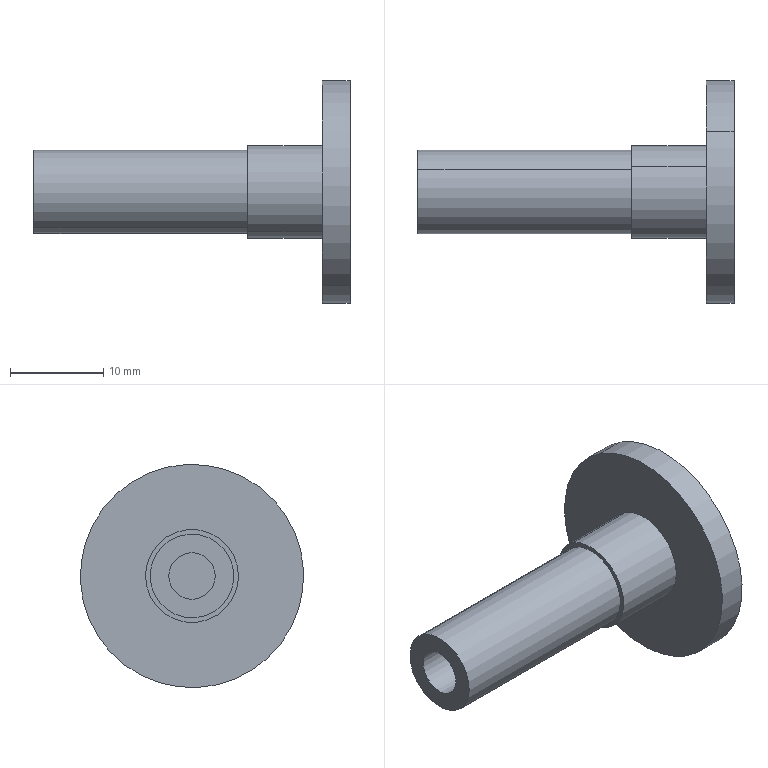Component | SolidWorks | FixedRotatingShaft-2 | 1 solid | 13 faces | box 34 x 24 x 24 mm | volume 3213 mm3 | cylinder 8 | plane 5 | commonest cylinder face diameters 5 x2 9 x2 10 x2 24 x2
STEP:
#1=CARTESIAN_POINT('',(-8.701,0.7338,14.898));
#2=VERTEX_POINT('',#1);
#3=CARTESIAN_POINT('',(-8.701,0.841,15.063));
#4=VERTEX_POINT('',#3);
#5=CARTESIAN_POINT('',(-8.701,0.7874,14.98));
#6=DIRECTION('',(-1.,-0.,0.));
#7=DIRECTION('',(0.,0.5444,0.8388));
#8=AXIS2_PLACEMENT_3D('',#5,#6,#7);
#9=CIRCLE('',#8,0.09843);
#10=EDGE_CURVE('',#2,#4,#9,.T.);
#11=ORIENTED_EDGE('',*,*,#10,.F.);
#12=CARTESIAN_POINT('',(-9.173,0.7338,14.898));
#13=VERTEX_POINT('',#12);
#14=CARTESIAN_POINT('',(-8.701,0.7338,14.898));
#15=DIRECTION('',(-1.,-0.,0.));
#16=VECTOR('',#15,39.37);
#17=LINE('',#14,#16);
#18=EDGE_CURVE('',#2,#13,#17,.T.);
#19=ORIENTED_EDGE('',*,*,#18,.T.);
#20=CARTESIAN_POINT('',(-9.173,0.841,15.063));
#21=VERTEX_POINT('',#20);
#22=CARTESIAN_POINT('',(-9.173,0.7874,14.98));
#23=DIRECTION('',(-1.,-0.,0.));
#24=DIRECTION('',(0.,0.5444,0.8388));
#25=AXIS2_PLACEMENT_3D('',#22,#23,#24);
#26=CIRCLE('',#25,0.09843);
#27=EDGE_CURVE('',#13,#21,#26,.T.);
#28=ORIENTED_EDGE('',*,*,#27,.T.);
#29=CARTESIAN_POINT('',(-8.701,0.841,15.063));
#30=DIRECTION('',(-1.,-0.,0.));
#31=VECTOR('',#30,39.37);
#32=LINE('',#29,#31);
#33=EDGE_CURVE('',#4,#21,#32,.T.);
#34=ORIENTED_EDGE('',*,*,#33,.F.);
#35=EDGE_LOOP('',(#11,#19,#28,#34));
#36=FACE_OUTER_BOUND('',#35,.T.);
#37=CARTESIAN_POINT('',(-8.701,0.7874,14.98));
#38=DIRECTION('',(-1.,-0.,0.));
#39=DIRECTION('',(0.,0.5444,0.8388));
#40=AXIS2_PLACEMENT_3D('',#37,#38,#39);
#41=CYLINDRICAL_SURFACE('',#40,0.09843);
#42=ADVANCED_FACE('',(#36),#41,.F.);
#43=CARTESIAN_POINT('',(-8.268,0.6909,14.832));
#44=VERTEX_POINT('',#43);
#45=CARTESIAN_POINT('',(-8.268,0.8839,15.129));
#46=VERTEX_POINT('',#45);
#47=CARTESIAN_POINT('',(-8.268,0.7874,14.98));
#48=DIRECTION('',(1.,0.,-0.));
#49=DIRECTION('',(0.,-0.5444,-0.8388));
#50=AXIS2_PLACEMENT_3D('',#47,#48,#49);
#51=CIRCLE('',#50,0.1772);
#52=EDGE_CURVE('',#44,#46,#51,.T.);
#53=ORIENTED_EDGE('',*,*,#52,.F.);
#54=CARTESIAN_POINT('',(-9.173,0.6909,14.832));
#55=VERTEX_POINT('',#54);
#56=CARTESIAN_POINT('',(-8.228,0.6909,14.832));
#57=DIRECTION('',(-1.,-0.,0.));
#58=VECTOR('',#57,39.37);
#59=LINE('',#56,#58);
#60=EDGE_CURVE('',#44,#55,#59,.T.);
#61=ORIENTED_EDGE('',*,*,#60,.T.);
#62=CARTESIAN_POINT('',(-9.173,0.8839,15.129));
#63=VERTEX_POINT('',#62);
#64=CARTESIAN_POINT('',(-9.173,0.7874,14.98));
#65=DIRECTION('',(-1.,-0.,0.));
#66=DIRECTION('',(0.,0.5444,0.8388));
#67=AXIS2_PLACEMENT_3D('',#64,#65,#66);
#68=CIRCLE('',#67,0.1772);
#69=EDGE_CURVE('',#63,#55,#68,.T.);
#70=ORIENTED_EDGE('',*,*,#69,.F.);
#71=CARTESIAN_POINT('',(-8.228,0.8839,15.129));
#72=DIRECTION('',(-1.,-0.,0.));
#73=VECTOR('',#72,39.37);
#74=LINE('',#71,#73);
#75=EDGE_CURVE('',#46,#63,#74,.T.);
#76=ORIENTED_EDGE('',*,*,#75,.F.);
#77=EDGE_LOOP('',(#53,#61,#70,#76));
#78=FACE_OUTER_BOUND('',#77,.T.);
#79=CARTESIAN_POINT('',(-8.228,0.7874,14.98));
#80=DIRECTION('',(-1.,-0.,0.));
#81=DIRECTION('',(0.,0.5444,0.8388));
#82=AXIS2_PLACEMENT_3D('',#79,#80,#81);
#83=CYLINDRICAL_SURFACE('',#82,0.1772);
#84=ADVANCED_FACE('',(#78),#83,.T.);
#85=CARTESIAN_POINT('',(-8.268,0.6802,14.815));
#86=VERTEX_POINT('',#85);
#87=CARTESIAN_POINT('',(-8.268,0.8946,15.145));
#88=VERTEX_POINT('',#87);
#89=CARTESIAN_POINT('',(-8.268,0.7874,14.98));
#90=DIRECTION('',(1.,0.,-0.));
#91=DIRECTION('',(0.,-0.5444,-0.8388));
#92=AXIS2_PLACEMENT_3D('',#89,#90,#91);
#93=CIRCLE('',#92,0.1969);
#94=EDGE_CURVE('',#86,#88,#93,.T.);
#95=ORIENTED_EDGE('',*,*,#94,.T.);
#96=CARTESIAN_POINT('',(-7.953,0.8946,15.145));
#97=VERTEX_POINT('',#96);
#98=CARTESIAN_POINT('',(-9.173,0.8946,15.145));
#99=DIRECTION('',(1.,0.,-0.));
#100=VECTOR('',#99,39.37);
#101=LINE('',#98,#100);
#102=EDGE_CURVE('',#88,#97,#101,.T.);
#103=ORIENTED_EDGE('',*,*,#102,.T.);
#104=CARTESIAN_POINT('',(-7.953,0.6802,14.815));
#105=VERTEX_POINT('',#104);
#106=CARTESIAN_POINT('',(-7.953,0.7874,14.98));
#107=DIRECTION('',(-1.,-0.,0.));
#108=DIRECTION('',(0.,0.5444,0.8388));
#109=AXIS2_PLACEMENT_3D('',#106,#107,#108);
#110=CIRCLE('',#109,0.1969);
#111=EDGE_CURVE('',#97,#105,#110,.T.);
#112=ORIENTED_EDGE('',*,*,#111,.T.);
#113=CARTESIAN_POINT('',(-9.173,0.6802,14.815));
#114=DIRECTION('',(1.,0.,-0.));
#115=VECTOR('',#114,39.37);
#116=LINE('',#113,#115);
#117=EDGE_CURVE('',#86,#105,#116,.T.);
#118=ORIENTED_EDGE('',*,*,#117,.F.);
#119=EDGE_LOOP('',(#95,#103,#112,#118));
#120=FACE_OUTER_BOUND('',#119,.T.);
#121=CARTESIAN_POINT('',(-9.173,0.7874,14.98));
#122=DIRECTION('',(1.,0.,-0.));
#123=DIRECTION('',(0.,-0.5444,-0.8388));
#124=AXIS2_PLACEMENT_3D('',#121,#122,#123);
#125=CYLINDRICAL_SURFACE('',#124,0.1969);
#126=ADVANCED_FACE('',(#120),#125,.T.);
#127=CARTESIAN_POINT('',(-7.953,1.045,15.377));
#128=VERTEX_POINT('',#127);
#129=CARTESIAN_POINT('',(-7.953,0.5302,14.584));
#130=VERTEX_POINT('',#129);
#131=CARTESIAN_POINT('',(-7.953,0.7874,14.98));
#132=DIRECTION('',(-1.,-0.,0.));
#133=DIRECTION('',(0.,0.5444,0.8388));
#134=AXIS2_PLACEMENT_3D('',#131,#132,#133);
#135=CIRCLE('',#134,0.4724);
#136=EDGE_CURVE('',#128,#130,#135,.T.);
#137=ORIENTED_EDGE('',*,*,#136,.F.);
#138=CARTESIAN_POINT('',(-7.835,1.045,15.377));
#139=VERTEX_POINT('',#138);
#140=CARTESIAN_POINT('',(-7.953,1.045,15.377));
#141=DIRECTION('',(1.,0.,-0.));
#142=VECTOR('',#141,39.37);
#143=LINE('',#140,#142);
#144=EDGE_CURVE('',#128,#139,#143,.T.);
#145=ORIENTED_EDGE('',*,*,#144,.T.);
#146=CARTESIAN_POINT('',(-7.835,0.5302,14.584));
#147=VERTEX_POINT('',#146);
#148=CARTESIAN_POINT('',(-7.835,0.7874,14.98));
#149=DIRECTION('',(-1.,-0.,0.));
#150=DIRECTION('',(0.,0.5444,0.8388));
#151=AXIS2_PLACEMENT_3D('',#148,#149,#150);
#152=CIRCLE('',#151,0.4724);
#153=EDGE_CURVE('',#139,#147,#152,.T.);
#154=ORIENTED_EDGE('',*,*,#153,.T.);
#155=CARTESIAN_POINT('',(-7.953,0.5302,14.584));
#156=DIRECTION('',(1.,0.,-0.));
#157=VECTOR('',#156,39.37);
#158=LINE('',#155,#157);
#159=EDGE_CURVE('',#130,#147,#158,.T.);
#160=ORIENTED_EDGE('',*,*,#159,.F.);
#161=EDGE_LOOP('',(#137,#145,#154,#160));
#162=FACE_OUTER_BOUND('',#161,.T.);
#163=CARTESIAN_POINT('',(-7.953,0.7874,14.98));
#164=DIRECTION('',(1.,0.,-0.));
#165=DIRECTION('',(0.,-0.5444,-0.8388));
#166=AXIS2_PLACEMENT_3D('',#163,#164,#165);
#167=CYLINDRICAL_SURFACE('',#166,0.4724);
#168=ADVANCED_FACE('',(#162),#167,.T.);
#169=CARTESIAN_POINT('',(-7.953,0.7874,14.98));
#170=DIRECTION('',(-1.,-0.,0.));
#171=DIRECTION('',(0.,0.5444,0.8388));
#172=AXIS2_PLACEMENT_3D('',#169,#170,#171);
#173=CIRCLE('',#172,0.4724);
#174=EDGE_CURVE('',#130,#128,#173,.T.);
#175=ORIENTED_EDGE('',*,*,#174,.T.);
#176=ORIENTED_EDGE('',*,*,#136,.T.);
#177=EDGE_LOOP('',(#175,#176));
#178=FACE_OUTER_BOUND('',#177,.T.);
#179=CARTESIAN_POINT('',(-7.953,0.7874,14.98));
#180=DIRECTION('',(-1.,-0.,0.));
#181=DIRECTION('',(0.,0.5444,0.8388));
#182=AXIS2_PLACEMENT_3D('',#179,#180,#181);
#183=CIRCLE('',#182,0.1969);
#184=EDGE_CURVE('',#105,#97,#183,.T.);
#185=ORIENTED_EDGE('',*,*,#184,.F.);
#186=ORIENTED_EDGE('',*,*,#111,.F.);
#187=EDGE_LOOP('',(#185,#186));
#188=FACE_BOUND('',#187,.T.);
#189=CARTESIAN_POINT('',(-7.953,0.7874,14.98));
#190=DIRECTION('',(-1.,-0.,0.));
#191=DIRECTION('',(-0.,0.5444,0.8388));
#192=AXIS2_PLACEMENT_3D('',#189,#190,#191);
#193=PLANE('',#192);
#194=ADVANCED_FACE('',(#178,#188),#193,.T.);
#195=ORIENTED_EDGE('',*,*,#144,.F.);
#196=ORIENTED_EDGE('',*,*,#174,.F.);
#197=ORIENTED_EDGE('',*,*,#159,.T.);
#198=CARTESIAN_POINT('',(-7.835,0.7874,14.98));
#199=DIRECTION('',(-1.,-0.,0.));
#200=DIRECTION('',(0.,0.5444,0.8388));
#201=AXIS2_PLACEMENT_3D('',#198,#199,#200);
#202=CIRCLE('',#201,0.4724);
#203=EDGE_CURVE('',#147,#139,#202,.T.);
#204=ORIENTED_EDGE('',*,*,#203,.T.);
#205=EDGE_LOOP('',(#195,#196,#197,#204));
#206=FACE_OUTER_BOUND('',#205,.T.);
#207=CARTESIAN_POINT('',(-7.953,0.7874,14.98));
#208=DIRECTION('',(1.,0.,-0.));
#209=DIRECTION('',(0.,-0.5444,-0.8388));
#210=AXIS2_PLACEMENT_3D('',#207,#208,#209);
#211=CYLINDRICAL_SURFACE('',#210,0.4724);
#212=ADVANCED_FACE('',(#206),#211,.T.);
#213=ORIENTED_EDGE('',*,*,#203,.F.);
#214=ORIENTED_EDGE('',*,*,#153,.F.);
#215=EDGE_LOOP('',(#213,#214));
#216=FACE_OUTER_BOUND('',#215,.T.);
#217=CARTESIAN_POINT('',(-7.835,0.7874,14.98));
#218=DIRECTION('',(-1.,-0.,0.));
#219=DIRECTION('',(-0.,0.5444,0.8388));
#220=AXIS2_PLACEMENT_3D('',#217,#218,#219);
#221=PLANE('',#220);
#222=ADVANCED_FACE('',(#216),#221,.F.);
#223=ORIENTED_EDGE('',*,*,#102,.F.);
#224=CARTESIAN_POINT('',(-8.268,0.7874,14.98));
#225=DIRECTION('',(1.,0.,-0.));
#226=DIRECTION('',(0.,-0.5444,-0.8388));
#227=AXIS2_PLACEMENT_3D('',#224,#225,#226);
#228=CIRCLE('',#227,0.1969);
#229=EDGE_CURVE('',#88,#86,#228,.T.);
#230=ORIENTED_EDGE('',*,*,#229,.T.);
#231=ORIENTED_EDGE('',*,*,#117,.T.);
#232=ORIENTED_EDGE('',*,*,#184,.T.);
#233=EDGE_LOOP('',(#223,#230,#231,#232));
#234=FACE_OUTER_BOUND('',#233,.T.);
#235=CARTESIAN_POINT('',(-9.173,0.7874,14.98));
#236=DIRECTION('',(1.,0.,-0.));
#237=DIRECTION('',(0.,-0.5444,-0.8388));
#238=AXIS2_PLACEMENT_3D('',#235,#236,#237);
#239=CYLINDRICAL_SURFACE('',#238,0.1969);
#240=ADVANCED_FACE('',(#234),#239,.T.);
#241=CARTESIAN_POINT('',(-8.268,0.7874,14.98));
#242=DIRECTION('',(1.,0.,-0.));
#243=DIRECTION('',(0.,-0.5444,-0.8388));
#244=AXIS2_PLACEMENT_3D('',#241,#242,#243);
#245=CIRCLE('',#244,0.1772);
#246=EDGE_CURVE('',#46,#44,#245,.T.);
#247=ORIENTED_EDGE('',*,*,#246,.T.);
#248=ORIENTED_EDGE('',*,*,#52,.T.);
#249=EDGE_LOOP('',(#247,#248));
#250=FACE_BOUND('',#249,.T.);
#251=ORIENTED_EDGE('',*,*,#94,.F.);
#252=ORIENTED_EDGE('',*,*,#229,.F.);
#253=EDGE_LOOP('',(#251,#252));
#254=FACE_OUTER_BOUND('',#253,.T.);
#255=CARTESIAN_POINT('',(-8.268,0.7874,14.98));
#256=DIRECTION('',(1.,0.,-0.));
#257=DIRECTION('',(0.,-0.5444,-0.8388));
#258=AXIS2_PLACEMENT_3D('',#255,#256,#257);
#259=PLANE('',#258);
#260=ADVANCED_FACE('',(#250,#254),#259,.F.);
#261=ORIENTED_EDGE('',*,*,#60,.F.);
#262=ORIENTED_EDGE('',*,*,#246,.F.);
#263=ORIENTED_EDGE('',*,*,#75,.T.);
#264=CARTESIAN_POINT('',(-9.173,0.7874,14.98));
#265=DIRECTION('',(-1.,-0.,0.));
#266=DIRECTION('',(0.,0.5444,0.8388));
#267=AXIS2_PLACEMENT_3D('',#264,#265,#266);
#268=CIRCLE('',#267,0.1772);
#269=EDGE_CURVE('',#55,#63,#268,.T.);
#270=ORIENTED_EDGE('',*,*,#269,.F.);
#271=EDGE_LOOP('',(#261,#262,#263,#270));
#272=FACE_OUTER_BOUND('',#271,.T.);
#273=CARTESIAN_POINT('',(-8.228,0.7874,14.98));
#274=DIRECTION('',(-1.,-0.,0.));
#275=DIRECTION('',(0.,0.5444,0.8388));
#276=AXIS2_PLACEMENT_3D('',#273,#274,#275);
#277=CYLINDRICAL_SURFACE('',#276,0.1772);
#278=ADVANCED_FACE('',(#272),#277,.T.);
#279=CARTESIAN_POINT('',(-8.701,0.7874,14.98));
#280=DIRECTION('',(-1.,-0.,0.));
#281=DIRECTION('',(0.,0.5444,0.8388));
#282=AXIS2_PLACEMENT_3D('',#279,#280,#281);
#283=CIRCLE('',#282,0.09843);
#284=EDGE_CURVE('',#4,#2,#283,.T.);
#285=ORIENTED_EDGE('',*,*,#284,.T.);
#286=ORIENTED_EDGE('',*,*,#10,.T.);
#287=EDGE_LOOP('',(#285,#286));
#288=FACE_OUTER_BOUND('',#287,.T.);
#289=CARTESIAN_POINT('',(-8.701,0.7874,14.98));
#290=DIRECTION('',(-1.,-0.,0.));
#291=DIRECTION('',(-0.,0.5444,0.8388));
#292=AXIS2_PLACEMENT_3D('',#289,#290,#291);
#293=PLANE('',#292);
#294=ADVANCED_FACE('',(#288),#293,.T.);
#295=ORIENTED_EDGE('',*,*,#18,.F.);
#296=ORIENTED_EDGE('',*,*,#284,.F.);
#297=ORIENTED_EDGE('',*,*,#33,.T.);
#298=CARTESIAN_POINT('',(-9.173,0.7874,14.98));
#299=DIRECTION('',(-1.,-0.,0.));
#300=DIRECTION('',(0.,0.5444,0.8388));
#301=AXIS2_PLACEMENT_3D('',#298,#299,#300);
#302=CIRCLE('',#301,0.09843);
#303=EDGE_CURVE('',#21,#13,#302,.T.);
#304=ORIENTED_EDGE('',*,*,#303,.T.);
#305=EDGE_LOOP('',(#295,#296,#297,#304));
#306=FACE_OUTER_BOUND('',#305,.T.);
#307=CARTESIAN_POINT('',(-8.701,0.7874,14.98));
#308=DIRECTION('',(-1.,-0.,0.));
#309=DIRECTION('',(0.,0.5444,0.8388));
#310=AXIS2_PLACEMENT_3D('',#307,#308,#309);
#311=CYLINDRICAL_SURFACE('',#310,0.09843);
#312=ADVANCED_FACE('',(#306),#311,.F.);
#313=ORIENTED_EDGE('',*,*,#303,.F.);
#314=ORIENTED_EDGE('',*,*,#27,.F.);
#315=EDGE_LOOP('',(#313,#314));
#316=FACE_BOUND('',#315,.T.);
#317=ORIENTED_EDGE('',*,*,#69,.T.);
#318=ORIENTED_EDGE('',*,*,#269,.T.);
#319=EDGE_LOOP('',(#317,#318));
#320=FACE_OUTER_BOUND('',#319,.T.);
#321=CARTESIAN_POINT('',(-9.173,0.7874,14.98));
#322=DIRECTION('',(-1.,-0.,0.));
#323=DIRECTION('',(-0.,0.5444,0.8388));
#324=AXIS2_PLACEMENT_3D('',#321,#322,#323);
#325=PLANE('',#324);
#326=ADVANCED_FACE('',(#316,#320),#325,.T.);
#327=CLOSED_SHELL('',(#42,#84,#126,#168,#194,#212,#222,#240,#260,#278,#294,#312,#326));
#328=MANIFOLD_SOLID_BREP('',#327);
#329=CARTESIAN_POINT('',(0.,0.,0.));
#330=DIRECTION('',(0.,0.,1.));
#331=DIRECTION('',(1.,0.,0.));
#332=AXIS2_PLACEMENT_3D('',#329,#330,#331);
#333=(LENGTH_UNIT()NAMED_UNIT(*)SI_UNIT($,.METRE.));
#334=LENGTH_MEASURE_WITH_UNIT(LENGTH_MEASURE(0.0254),#333);
#335=DIMENSIONAL_EXPONENTS(1.,0.,0.,0.,0.,0.,0.);
#336=(CONVERSION_BASED_UNIT('',#334)LENGTH_UNIT()NAMED_UNIT(#335));
#337=UNCERTAINTY_MEASURE_WITH_UNIT(LENGTH_MEASURE(0.00001),#336,'','');
#338=(NAMED_UNIT(*)PLANE_ANGLE_UNIT()SI_UNIT($,.RADIAN.));
#339=(NAMED_UNIT(*)SI_UNIT($,.STERADIAN.)SOLID_ANGLE_UNIT());
#340=(GEOMETRIC_REPRESENTATION_CONTEXT(3)GLOBAL_UNCERTAINTY_ASSIGNED_CONTEXT((#337))GLOBAL_UNIT_ASSIGNED_CONTEXT((#336,#338,#339))REPRESENTATION_CONTEXT('',''));
#341=ADVANCED_BREP_SHAPE_REPRESENTATION('',(#328,#332),#340);
#342=COLOUR_RGB('',0.7922,0.8196,0.9333);
#343=FILL_AREA_STYLE_COLOUR('',#342);
#344=FILL_AREA_STYLE('',(#343));
#345=SURFACE_STYLE_FILL_AREA(#344);
#346=SURFACE_SIDE_STYLE('',(#345));
#347=SURFACE_STYLE_USAGE(.BOTH.,#346);
#348=PRESENTATION_STYLE_ASSIGNMENT((#347));
#349=STYLED_ITEM('',(#348),#328);
#350=PRESENTATION_LAYER_ASSIGNMENT('','',(#349));
#351=(LENGTH_UNIT()NAMED_UNIT(*)SI_UNIT($,.METRE.));
#352=LENGTH_MEASURE_WITH_UNIT(LENGTH_MEASURE(0.0254),#351);
#353=DIMENSIONAL_EXPONENTS(1.,0.,0.,0.,0.,0.,0.);
#354=(CONVERSION_BASED_UNIT('',#352)LENGTH_UNIT()NAMED_UNIT(#353));
#355=UNCERTAINTY_MEASURE_WITH_UNIT(LENGTH_MEASURE(0.00001),#354,'','');
#356=(NAMED_UNIT(*)PLANE_ANGLE_UNIT()SI_UNIT($,.RADIAN.));
#357=(NAMED_UNIT(*)SI_UNIT($,.STERADIAN.)SOLID_ANGLE_UNIT());
#358=(GEOMETRIC_REPRESENTATION_CONTEXT(3)GLOBAL_UNCERTAINTY_ASSIGNED_CONTEXT((#355))GLOBAL_UNIT_ASSIGNED_CONTEXT((#354,#356,#357))REPRESENTATION_CONTEXT('',''));
#359=MECHANICAL_DESIGN_GEOMETRIC_PRESENTATION_REPRESENTATION('',(#349),#358);